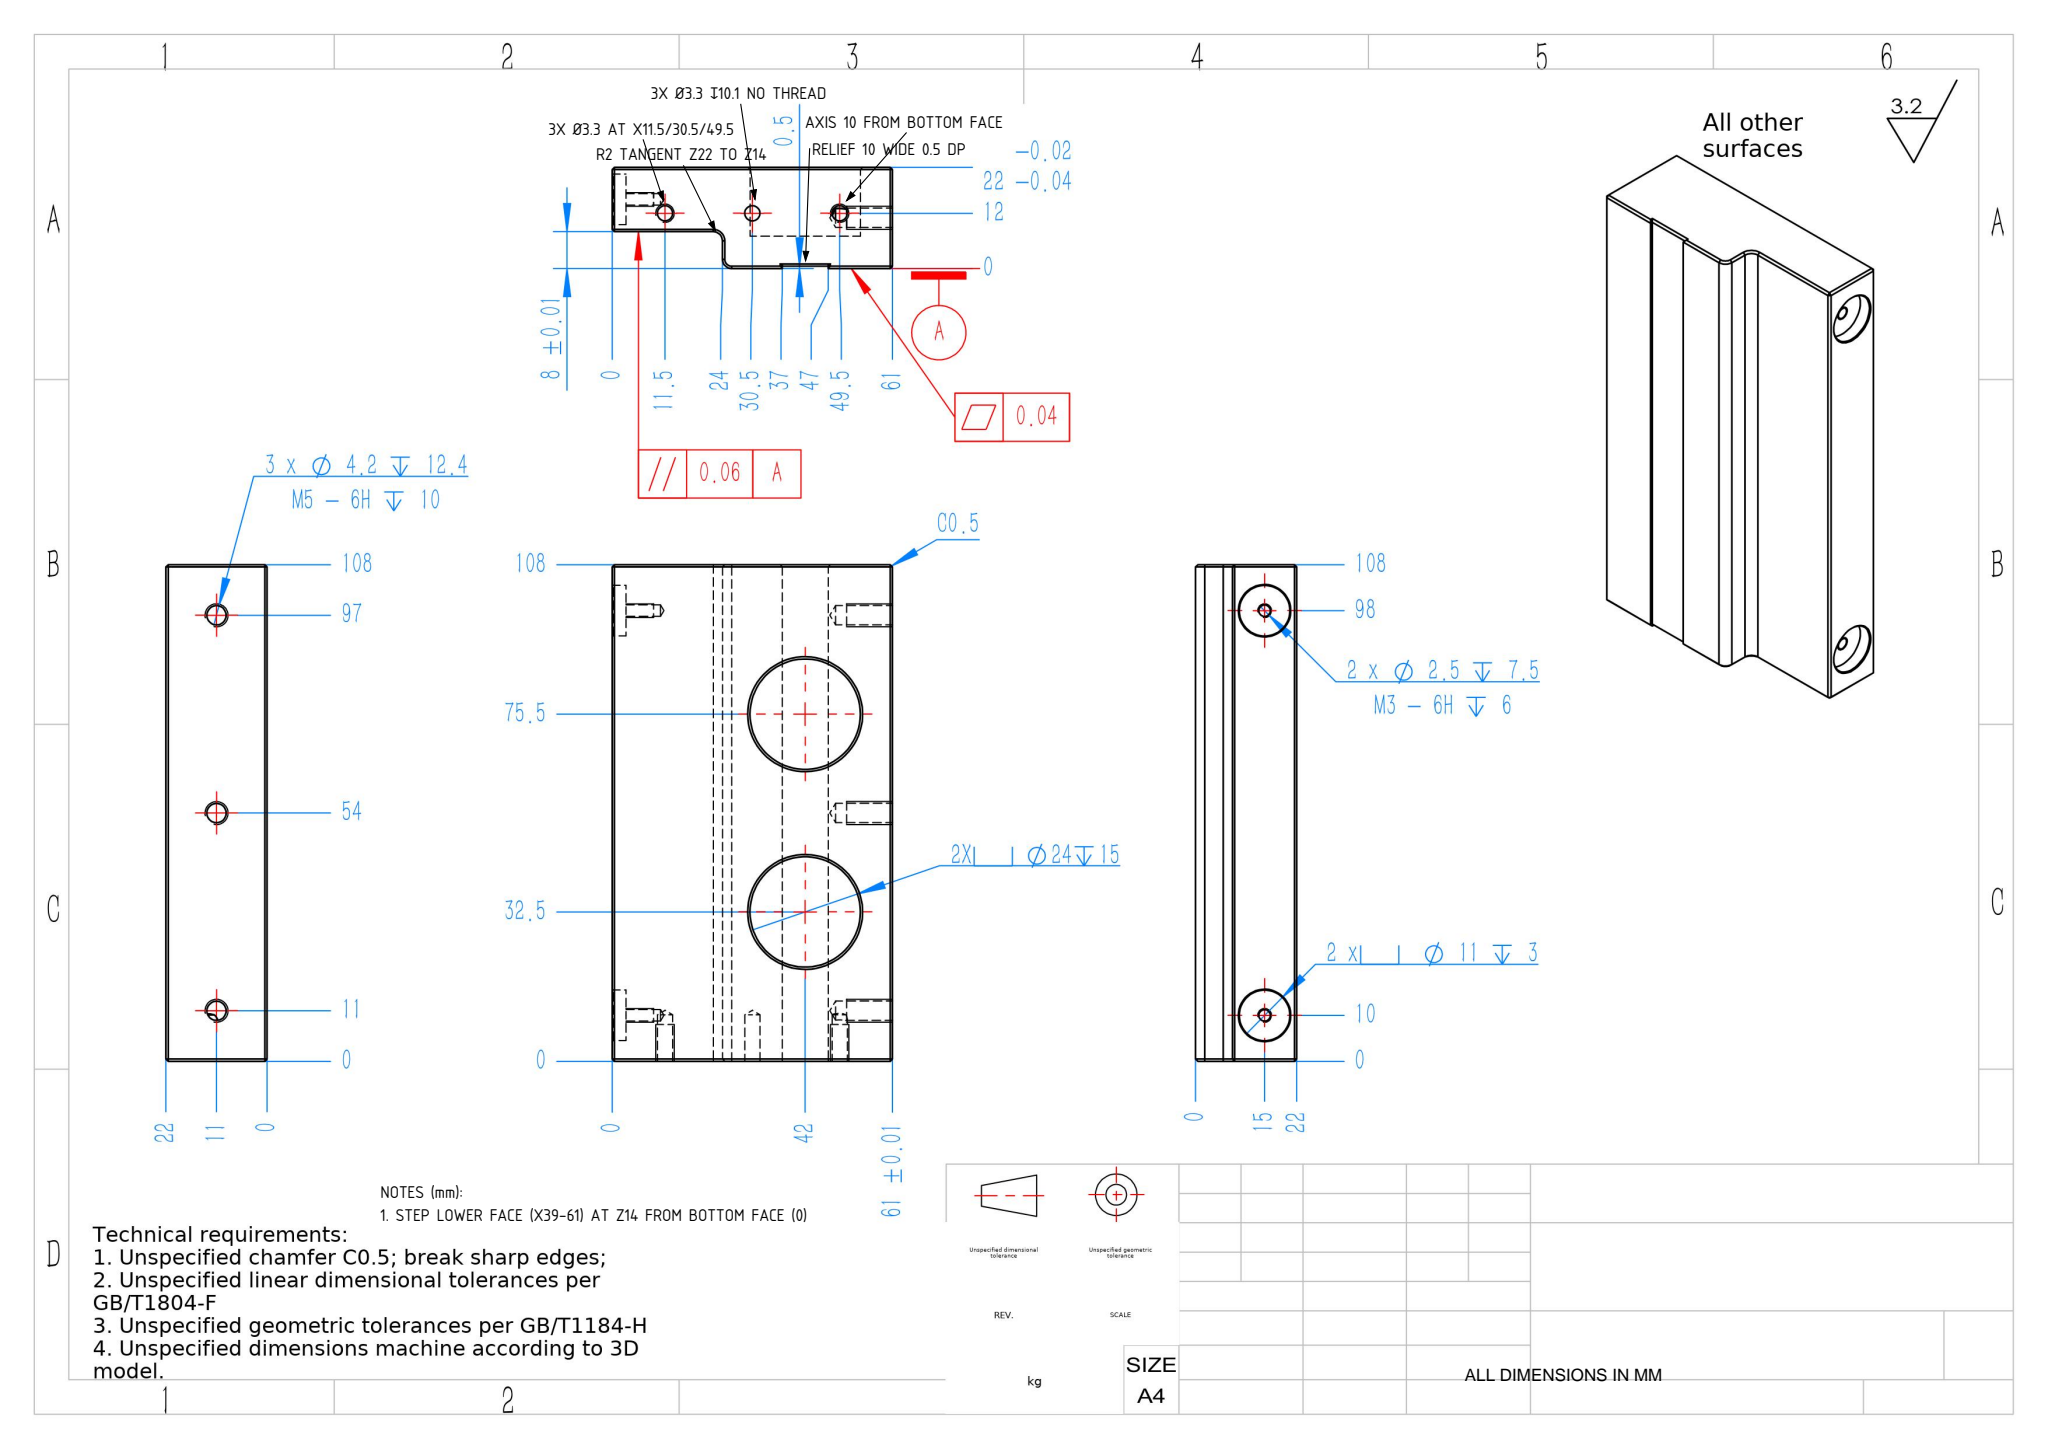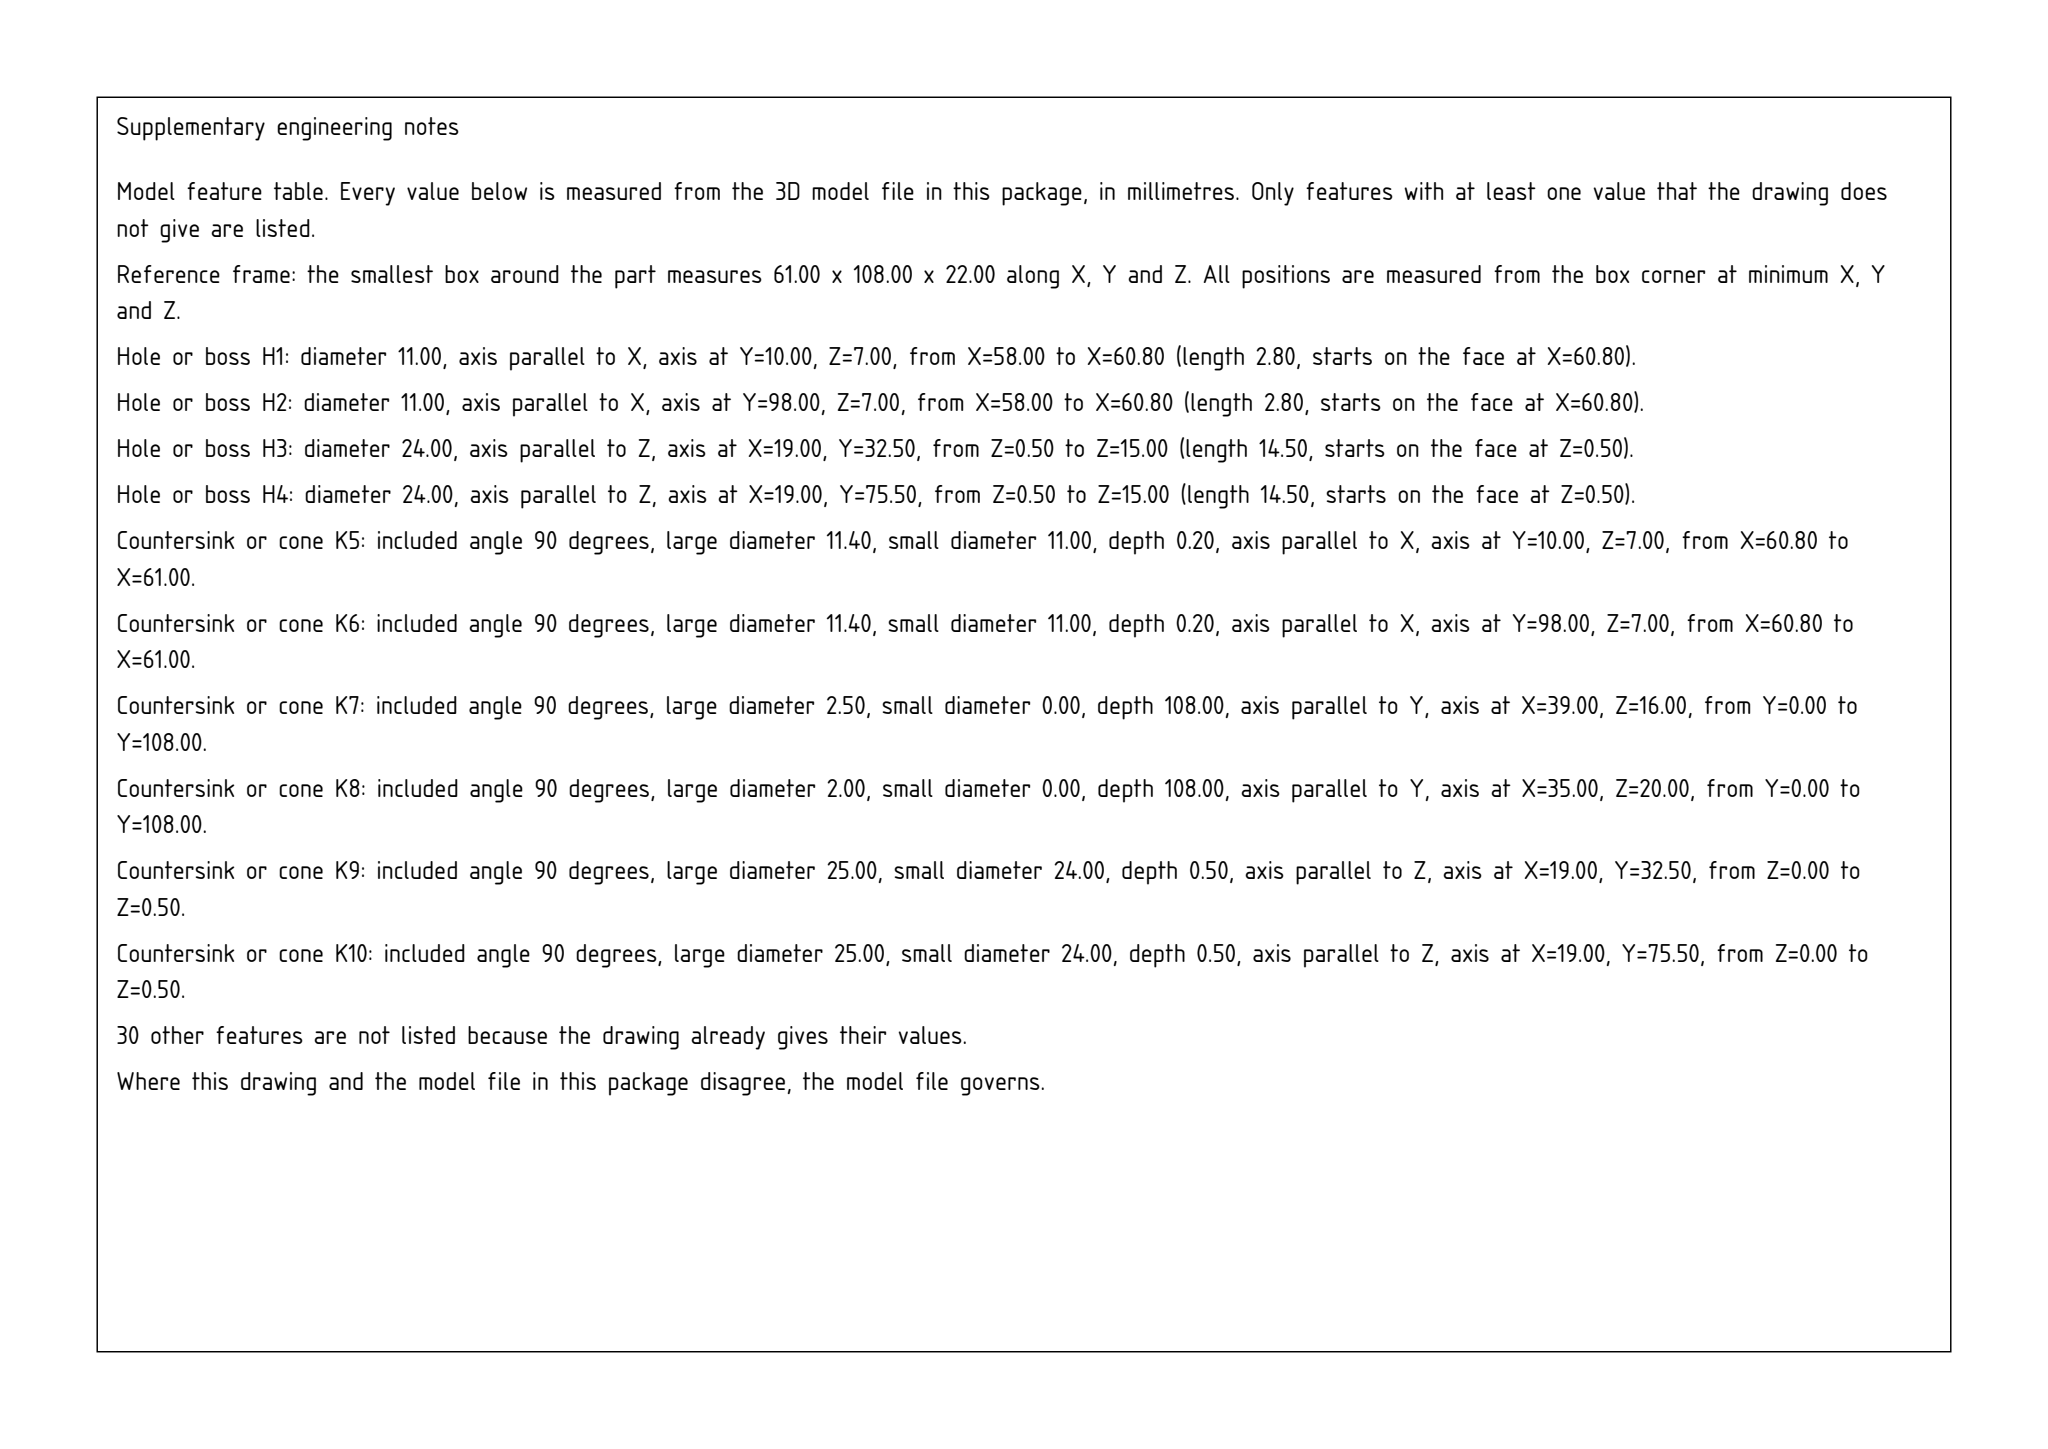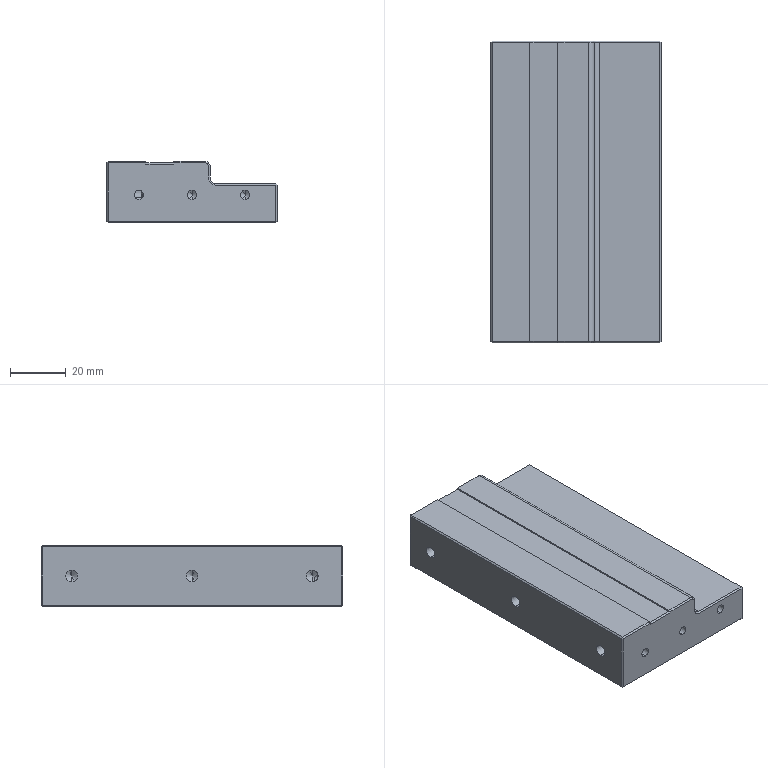Part | SolidWorks | mm | 1 solid | 100 faces | box 61 x 108 x 22 mm | volume 108535 mm3 | plane 46 | cone 28 | cylinder 26 | commonest cylinder face diameters 3.3 x6 4.2 x6 24 x4 2.5 x4 11 x4 4 x2
Drawing notes:
BLEND TANGENTS AT X35 (TOP Z22) AND X39 (LOWER FACE Z14) | from the solid: plane z=22 extent x [24,35]; plane z=14 extent x [39,60.5]
TOP FACE RELIEF X14 TO X24 (10 WIDE) 0.5 DP FROM Z22, FULL LGTH | from the solid: plane z=21.5 extent x [14,24], y [0.5,107.5]; planes x=14 & x=24 extent z [21,22]
3X Ø3.3 IN Y0 FACE, AT X11.5, X30.5, X49.5 | from the solid: hole/bore dia 3.3, axis y, axis_pos x=11.5/30.5/49.5, in plane y=0
3X Ø3.3 DP 10.1 PLAIN HOLE, NO THREAD | from the solid: hole/bore dia 3.3 axis y from 0.0 to 10.1; no tapped feature in STEP
3X Ø3.3 HOLE AXES AT Z10 FROM BOTTOM FACE (0) | from the solid: hole/bore dia 3.3 axis_pos z=10.0; bottom face plane z=0
STEP LOWER FACE (X39-61) AT Z14 FROM BOTTOM FACE (0) | from the solid: axis_plane z=14.0, extent x[39.0,60.5] y[0.5,107.5]